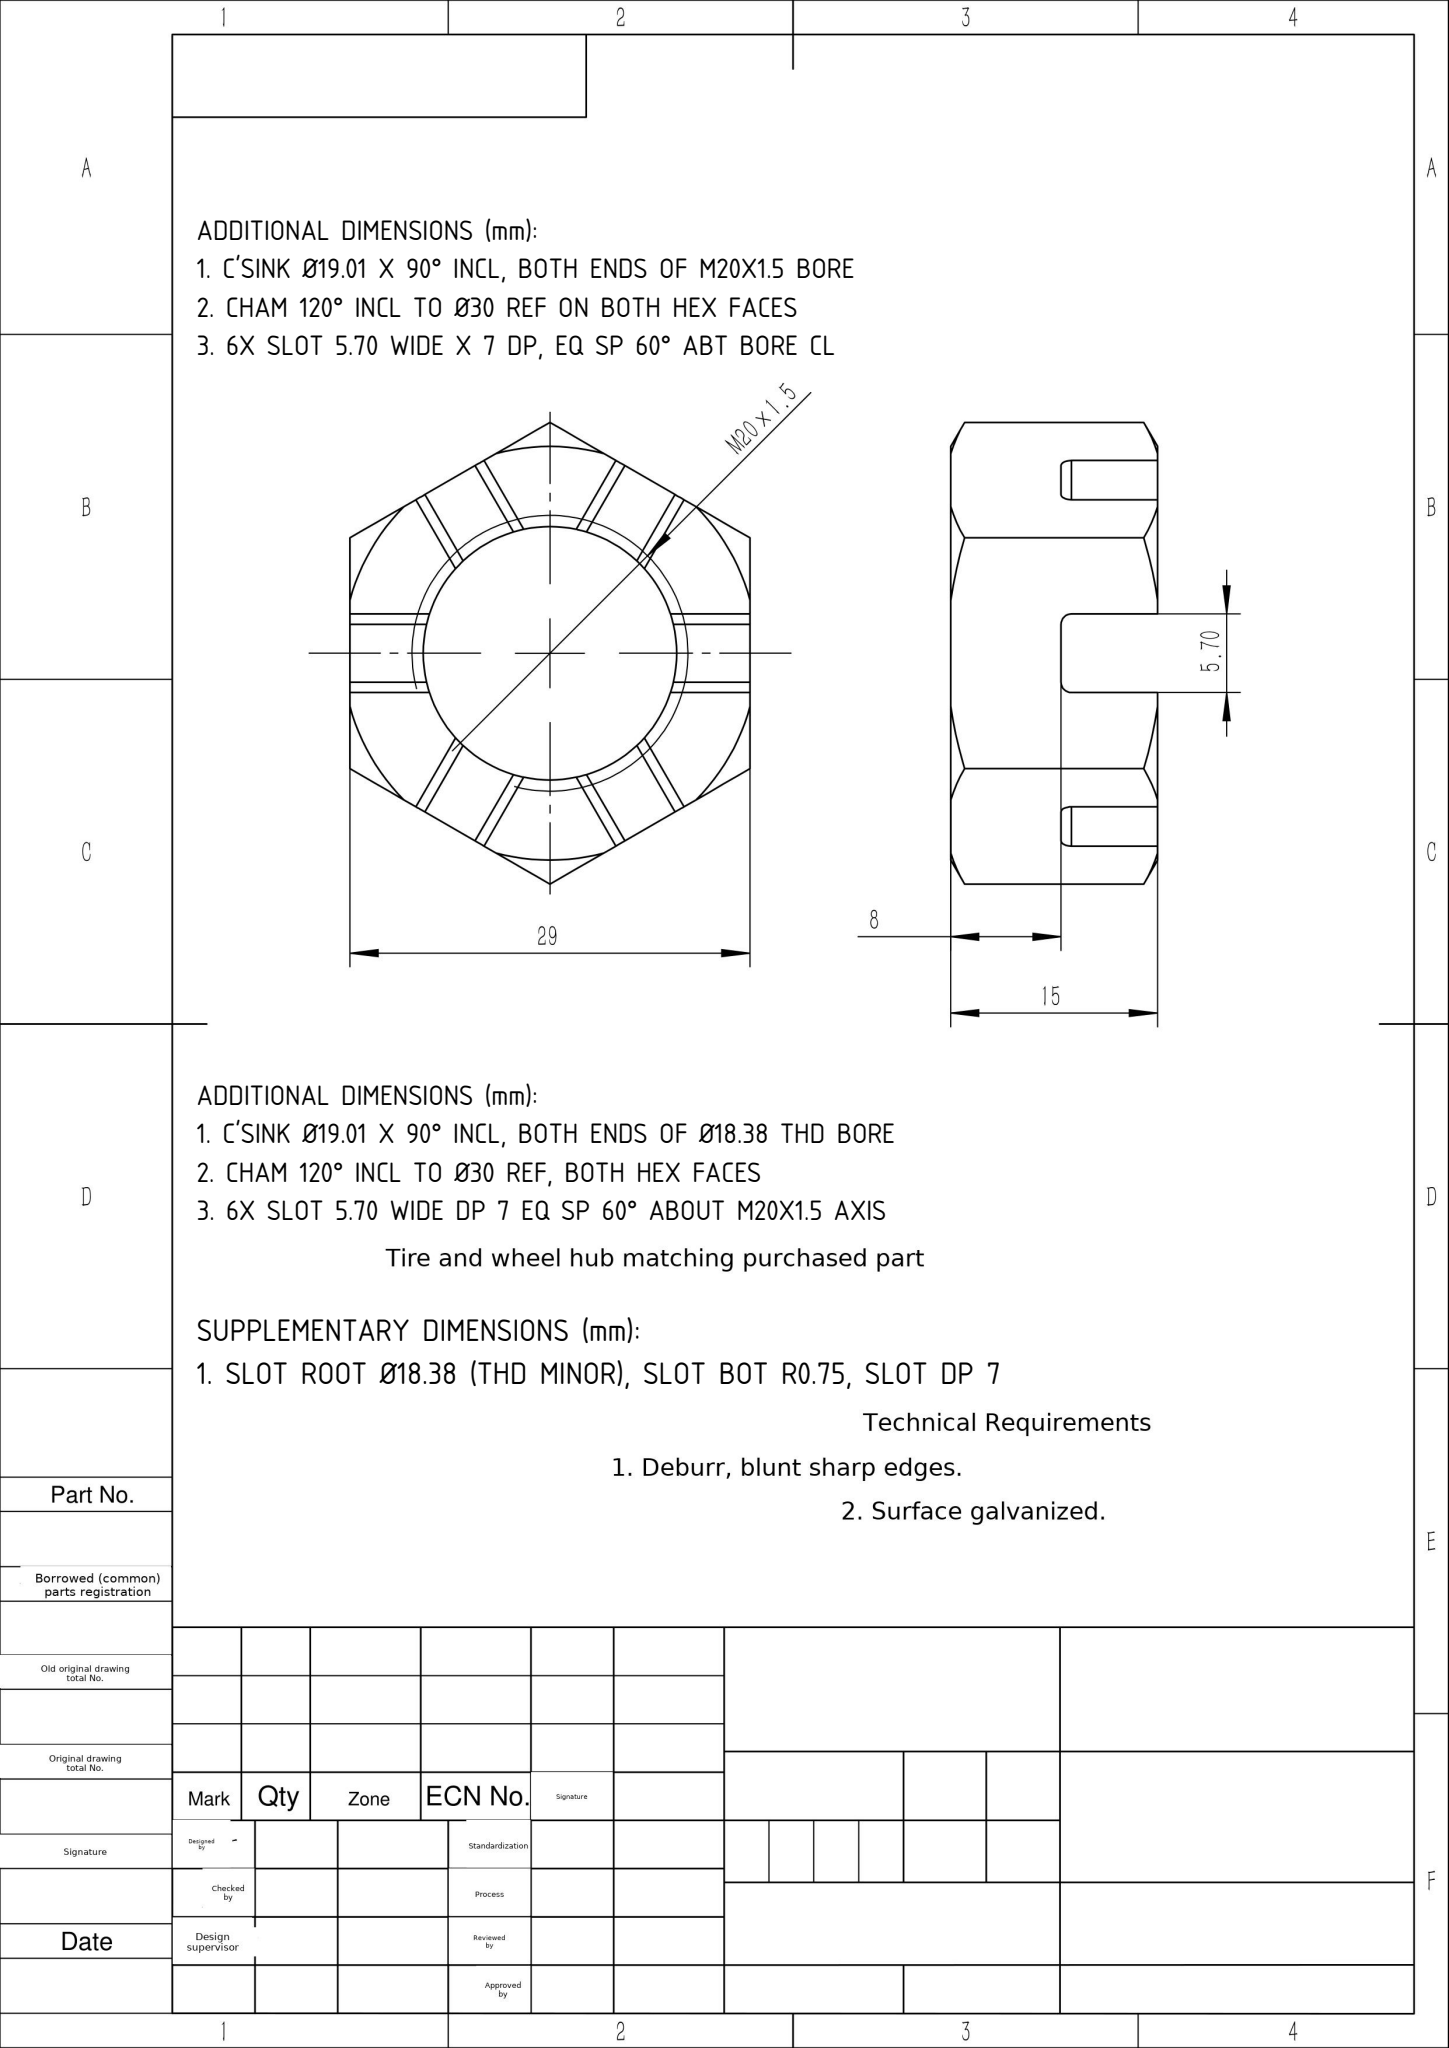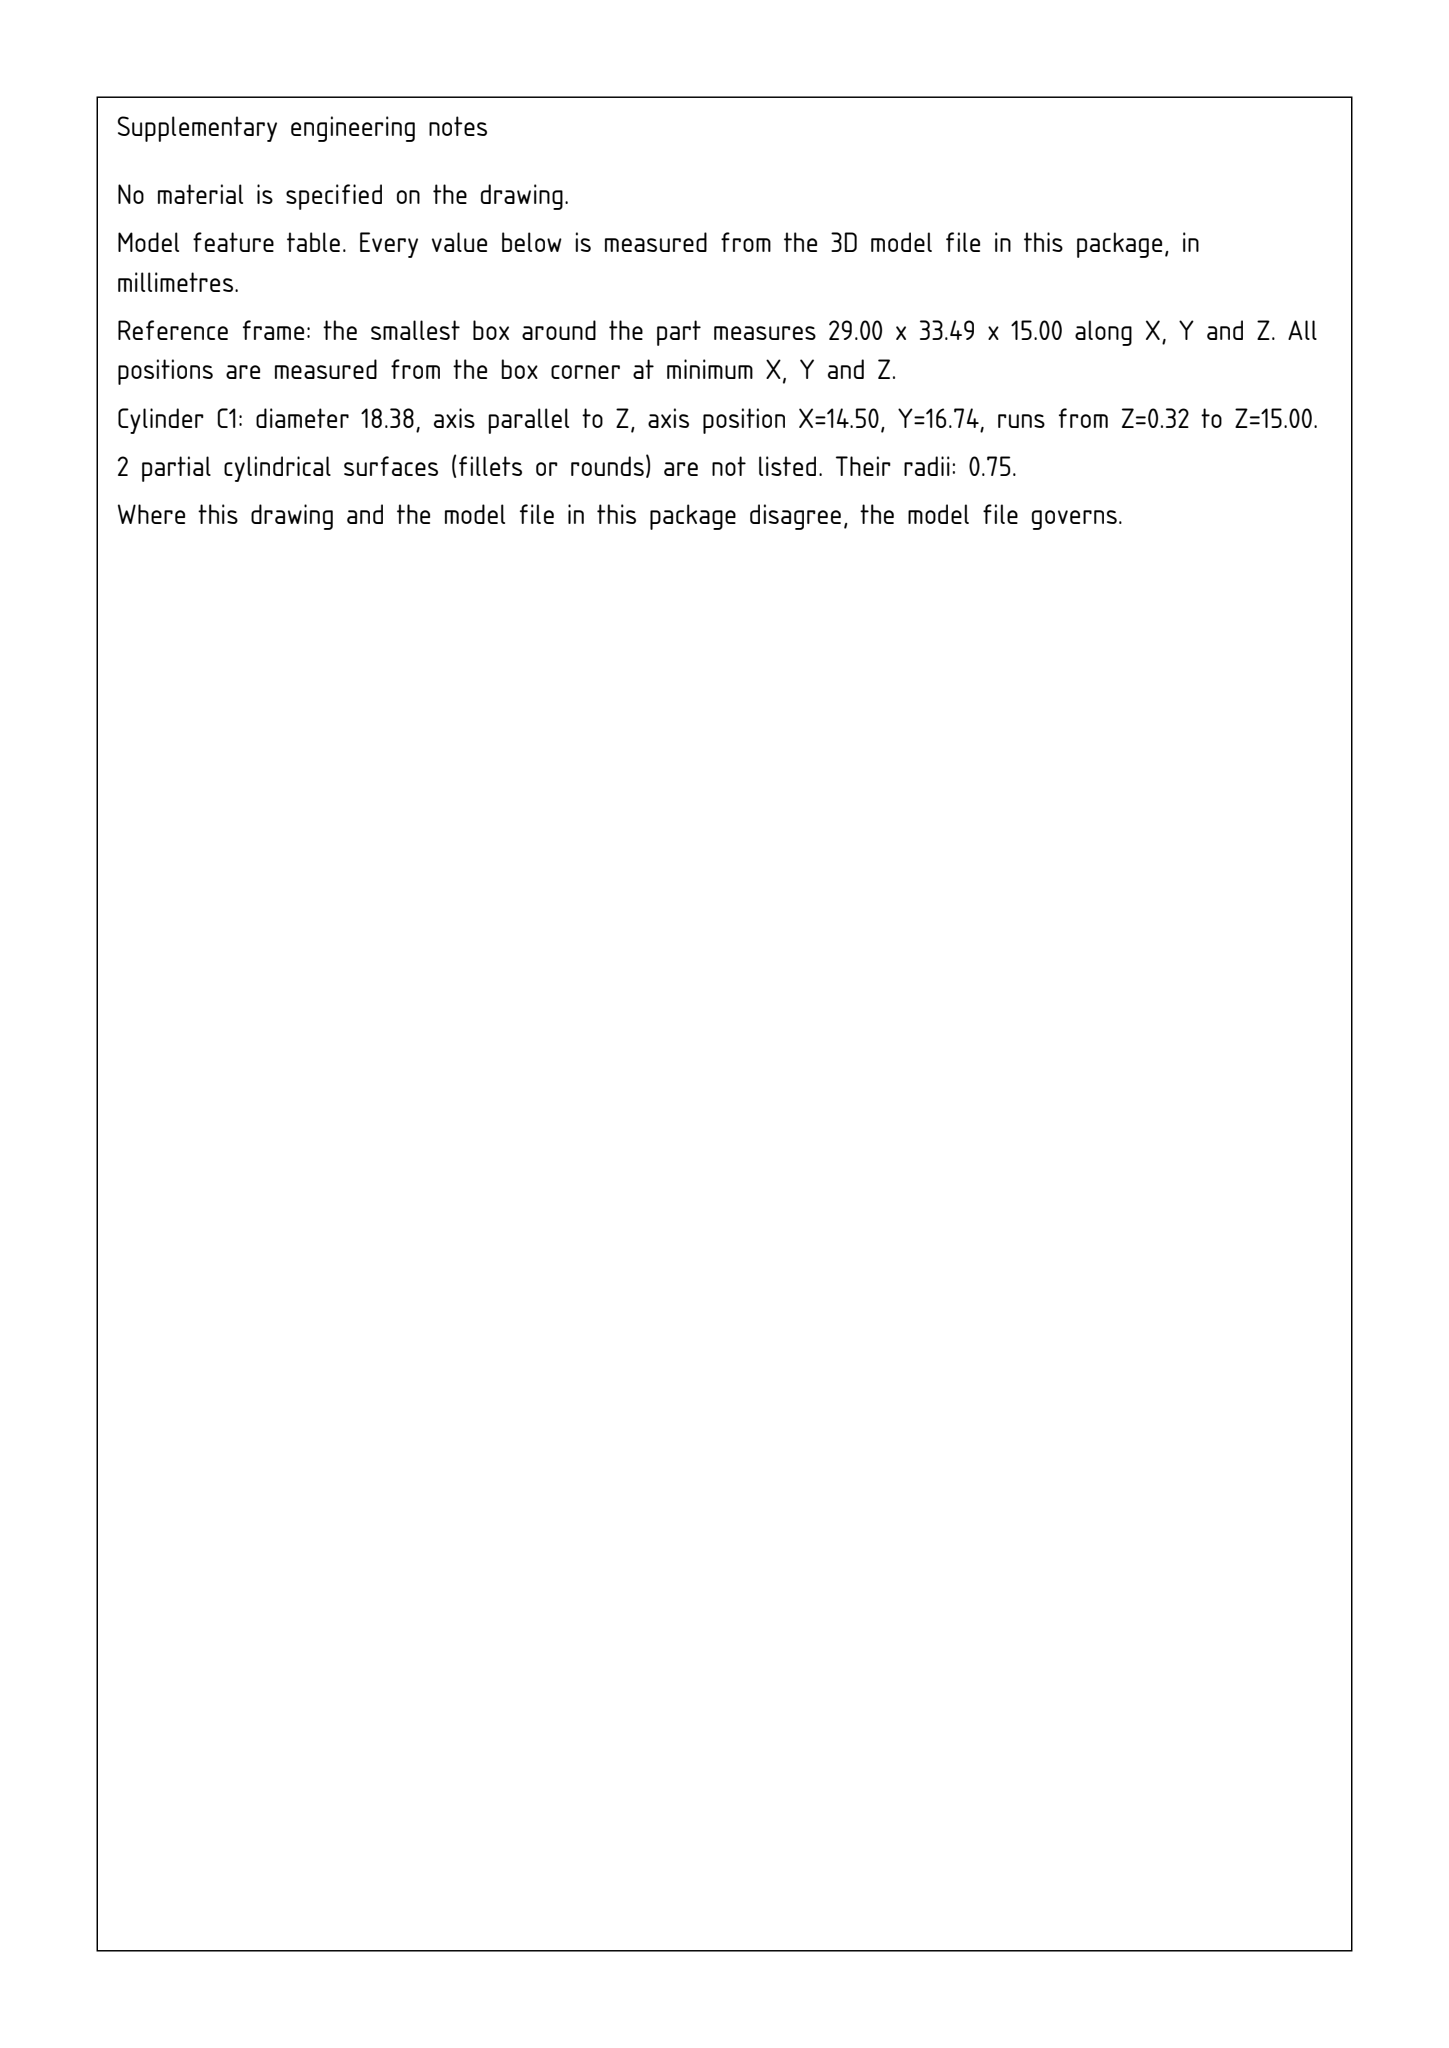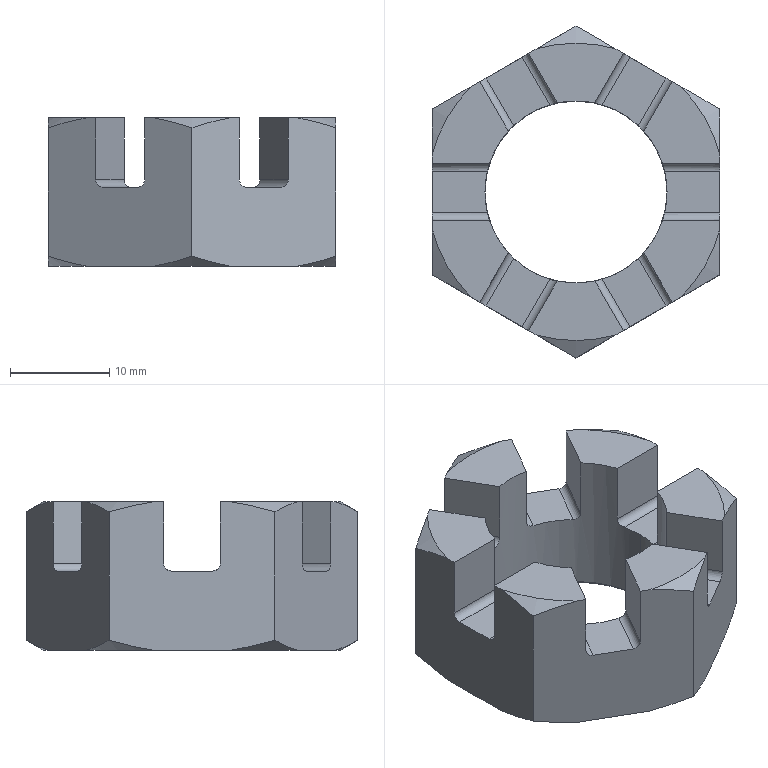Part | SolidWorks | mm | 1 solid | 59 faces | box 29 x 33.49 x 15 mm | volume 5621 mm3 | plane 31 | cone 14 | cylinder 14 | commonest cylinder face diameters 1.5 x12 18.376 x2